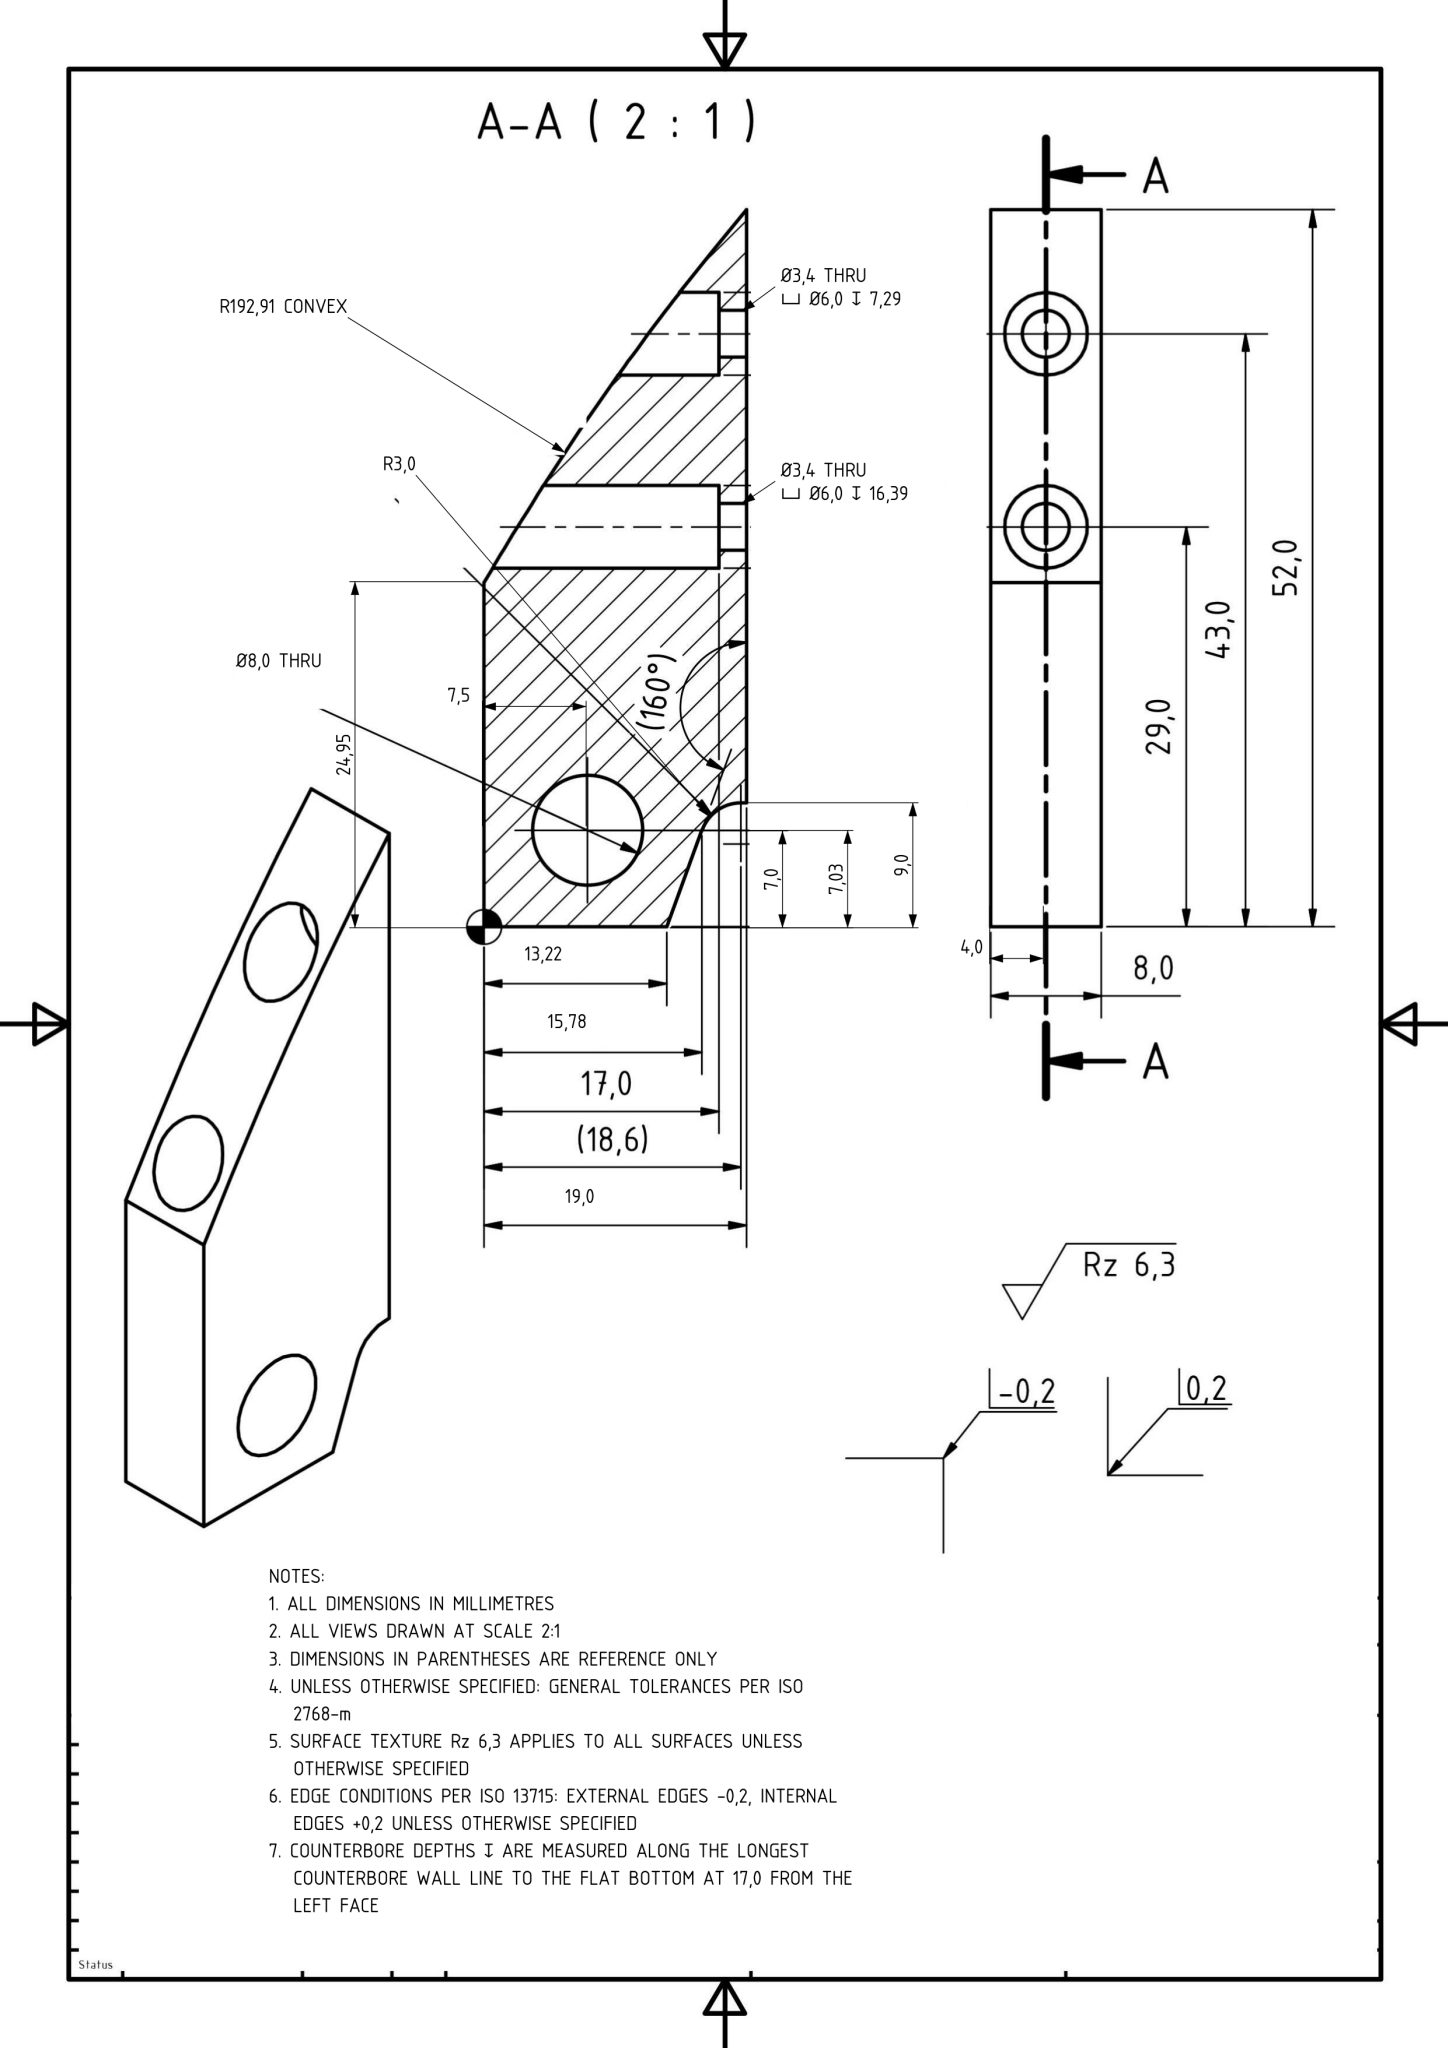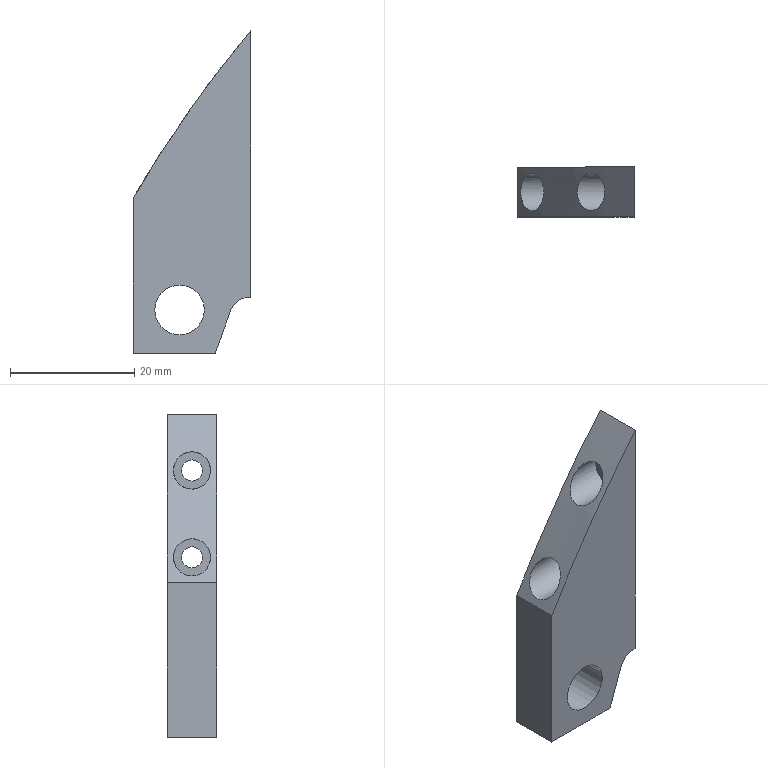Part | NX | mm | 1 solid | 16 faces | box 19 x 8 x 52 mm | volume 4687 mm3 | plane 9 | cylinder 7 | commonest cylinder face diameters 6 x3 3.4 x2 8 x1 385.82 x1
STEP:
#1=(LENGTH_UNIT()NAMED_UNIT(*)SI_UNIT(.MILLI.,.METRE.));
#2=UNCERTAINTY_MEASURE_WITH_UNIT(LENGTH_MEASURE(0.000001),#1,'','');
#3=(NAMED_UNIT(*)PLANE_ANGLE_UNIT()SI_UNIT($,.RADIAN.));
#4=PLANE_ANGLE_MEASURE_WITH_UNIT(PLANE_ANGLE_MEASURE(0.01745),#3);
#5=DIMENSIONAL_EXPONENTS(0.,0.,0.,0.,0.,0.,0.);
#6=(CONVERSION_BASED_UNIT('',#4)NAMED_UNIT(#5)PLANE_ANGLE_UNIT());
#7=(NAMED_UNIT(*)SI_UNIT($,.STERADIAN.)SOLID_ANGLE_UNIT());
#8=(GEOMETRIC_REPRESENTATION_CONTEXT(3)GLOBAL_UNCERTAINTY_ASSIGNED_CONTEXT((#2))GLOBAL_UNIT_ASSIGNED_CONTEXT((#6,#7,#1))REPRESENTATION_CONTEXT('',''));
#9=COLOUR_RGB('',0.898,0.9,0.9);
#10=FILL_AREA_STYLE_COLOUR('',#9);
#11=FILL_AREA_STYLE('',(#10));
#12=SURFACE_STYLE_FILL_AREA(#11);
#13=SURFACE_SIDE_STYLE('',(#12));
#14=SURFACE_STYLE_USAGE(.BOTH.,#13);
#15=PRESENTATION_STYLE_ASSIGNMENT((#14));
#16=CARTESIAN_POINT('',(-34.399,0.,-43.));
#17=VERTEX_POINT('',#16);
#18=CARTESIAN_POINT('',(-37.218,0.,-44.974));
#19=VERTEX_POINT('',#18);
#20=CARTESIAN_POINT('',(-34.399,0.,-46.));
#21=DIRECTION('',(0.,-1.,0.));
#22=DIRECTION('',(-0.5736,0.,0.8192));
#23=AXIS2_PLACEMENT_3D('',#20,#21,#22);
#24=CIRCLE('',#23,3.);
#25=EDGE_CURVE('',#17,#19,#24,.T.);
#26=ORIENTED_EDGE('',*,*,#25,.T.);
#27=CARTESIAN_POINT('',(-37.218,8.,-44.974));
#28=VERTEX_POINT('',#27);
#29=CARTESIAN_POINT('',(-37.218,0.,-44.974));
#30=DIRECTION('',(0.,1.,0.));
#31=VECTOR('',#30,8.);
#32=LINE('',#29,#31);
#33=EDGE_CURVE('',#19,#28,#32,.T.);
#34=ORIENTED_EDGE('',*,*,#33,.T.);
#35=CARTESIAN_POINT('',(-34.399,8.,-43.));
#36=VERTEX_POINT('',#35);
#37=CARTESIAN_POINT('',(-34.399,8.,-46.));
#38=DIRECTION('',(0.,1.,0.));
#39=DIRECTION('',(-0.5736,0.,0.8192));
#40=AXIS2_PLACEMENT_3D('',#37,#38,#39);
#41=CIRCLE('',#40,3.);
#42=EDGE_CURVE('',#28,#36,#41,.T.);
#43=ORIENTED_EDGE('',*,*,#42,.T.);
#44=CARTESIAN_POINT('',(-34.399,8.,-43.));
#45=DIRECTION('',(0.,-1.,0.));
#46=VECTOR('',#45,8.);
#47=LINE('',#44,#46);
#48=EDGE_CURVE('',#36,#17,#47,.T.);
#49=ORIENTED_EDGE('',*,*,#48,.T.);
#50=EDGE_LOOP('',(#26,#34,#43,#49));
#51=FACE_OUTER_BOUND('',#50,.T.);
#52=CARTESIAN_POINT('',(-34.399,0.,-46.));
#53=DIRECTION('',(0.,1.,0.));
#54=DIRECTION('',(-0.5736,0.,0.8192));
#55=AXIS2_PLACEMENT_3D('',#52,#53,#54);
#56=CYLINDRICAL_SURFACE('',#55,3.);
#57=ADVANCED_FACE('',(#51),#56,.F.);
#58=ORIENTED_EDGE('',*,*,#33,.F.);
#59=CARTESIAN_POINT('',(-39.776,0.,-52.));
#60=VERTEX_POINT('',#59);
#61=CARTESIAN_POINT('',(-37.218,0.,-44.974));
#62=DIRECTION('',(-0.342,0.,-0.9397));
#63=VECTOR('',#62,7.477);
#64=LINE('',#61,#63);
#65=EDGE_CURVE('',#19,#60,#64,.T.);
#66=ORIENTED_EDGE('',*,*,#65,.T.);
#67=CARTESIAN_POINT('',(-39.776,8.,-52.));
#68=VERTEX_POINT('',#67);
#69=CARTESIAN_POINT('',(-39.776,0.,-52.));
#70=DIRECTION('',(0.,1.,0.));
#71=VECTOR('',#70,8.);
#72=LINE('',#69,#71);
#73=EDGE_CURVE('',#60,#68,#72,.T.);
#74=ORIENTED_EDGE('',*,*,#73,.T.);
#75=CARTESIAN_POINT('',(-37.218,8.,-44.974));
#76=DIRECTION('',(-0.342,0.,-0.9397));
#77=VECTOR('',#76,7.477);
#78=LINE('',#75,#77);
#79=EDGE_CURVE('',#28,#68,#78,.T.);
#80=ORIENTED_EDGE('',*,*,#79,.F.);
#81=EDGE_LOOP('',(#58,#66,#74,#80));
#82=FACE_OUTER_BOUND('',#81,.T.);
#83=CARTESIAN_POINT('',(-36.5,0.,-43.));
#84=DIRECTION('',(0.9397,0.,-0.342));
#85=DIRECTION('',(-0.342,0.,-0.9397));
#86=AXIS2_PLACEMENT_3D('',#83,#84,#85);
#87=PLANE('',#86);
#88=ADVANCED_FACE('',(#82),#87,.T.);
#89=CARTESIAN_POINT('',(-43.29,4.,-12.));
#90=VERTEX_POINT('',#89);
#91=CARTESIAN_POINT('',(-43.29,4.,-12.));
#92=CARTESIAN_POINT('',(-43.29,4.373,-12.));
#93=CARTESIAN_POINT('',(-43.237,4.764,-11.926));
#94=CARTESIAN_POINT('',(-43.035,5.47,-11.643));
#95=CARTESIAN_POINT('',(-42.885,5.785,-11.435));
#96=CARTESIAN_POINT('',(-42.515,6.344,-10.92));
#97=CARTESIAN_POINT('',(-42.254,6.596,-10.56));
#98=CARTESIAN_POINT('',(-41.691,6.924,-9.79));
#99=CARTESIAN_POINT('',(-41.389,7.,-9.379));
#100=CARTESIAN_POINT('',(-40.822,7.,-8.616));
#101=CARTESIAN_POINT('',(-40.513,6.923,-8.203));
#102=CARTESIAN_POINT('',(-39.931,6.592,-7.432));
#103=CARTESIAN_POINT('',(-39.658,6.339,-7.073));
#104=CARTESIAN_POINT('',(-39.267,5.78,-6.563));
#105=CARTESIAN_POINT('',(-39.108,5.467,-6.356));
#106=CARTESIAN_POINT('',(-38.891,4.764,-6.074));
#107=CARTESIAN_POINT('',(-38.834,4.374,-6.));
#108=CARTESIAN_POINT('',(-38.834,3.626,-6.));
#109=CARTESIAN_POINT('',(-38.891,3.236,-6.074));
#110=CARTESIAN_POINT('',(-39.108,2.533,-6.356));
#111=CARTESIAN_POINT('',(-39.267,2.22,-6.563));
#112=CARTESIAN_POINT('',(-39.658,1.661,-7.073));
#113=CARTESIAN_POINT('',(-39.931,1.408,-7.432));
#114=CARTESIAN_POINT('',(-40.513,1.077,-8.203));
#115=CARTESIAN_POINT('',(-40.822,1.,-8.616));
#116=CARTESIAN_POINT('',(-41.389,1.,-9.379));
#117=CARTESIAN_POINT('',(-41.691,1.076,-9.79));
#118=CARTESIAN_POINT('',(-42.254,1.404,-10.56));
#119=CARTESIAN_POINT('',(-42.515,1.656,-10.92));
#120=CARTESIAN_POINT('',(-42.885,2.215,-11.435));
#121=CARTESIAN_POINT('',(-43.035,2.53,-11.643));
#122=CARTESIAN_POINT('',(-43.237,3.236,-11.926));
#123=CARTESIAN_POINT('',(-43.29,3.627,-12.));
#124=CARTESIAN_POINT('',(-43.29,4.,-12.));
#125=B_SPLINE_CURVE_WITH_KNOTS('',3,(#91,#92,#93,#94,#95,#96,#97,#98,#99,#100,#101,#102,#103,#104,#105,#106,#107,#108,#109,#110,#111,#112,#113,#114,#115,#116,#117,#118,#119,#120,#121,#122,#123,#124),.UNSPECIFIED.,.T.,.U.,(4,2,2,2,2,2,2,2,2,2,2,2,2,2,2,2,4),(0.,0.1119,0.2237,0.3655,0.5073,0.6507,0.7941,0.9062,1.018,1.13,1.243,1.386,1.529,1.671,1.813,1.925,2.037),.UNSPECIFIED.);
#126=EDGE_CURVE('',#90,#90,#125,.T.);
#127=ORIENTED_EDGE('',*,*,#126,.F.);
#128=EDGE_LOOP('',(#127));
#129=FACE_OUTER_BOUND('',#128,.T.);
#130=CARTESIAN_POINT('',(-36.,4.,-6.));
#131=VERTEX_POINT('',#130);
#132=CARTESIAN_POINT('',(-36.,4.,-9.));
#133=DIRECTION('',(1.,0.,0.));
#134=DIRECTION('',(0.,0.,-1.));
#135=AXIS2_PLACEMENT_3D('',#132,#133,#134);
#136=CIRCLE('',#135,3.);
#137=EDGE_CURVE('',#131,#131,#136,.T.);
#138=ORIENTED_EDGE('',*,*,#137,.T.);
#139=EDGE_LOOP('',(#138));
#140=FACE_BOUND('',#139,.T.);
#141=CARTESIAN_POINT('',(-53.,4.,-9.));
#142=DIRECTION('',(1.,0.,-0.));
#143=DIRECTION('',(0.,0.,-1.));
#144=AXIS2_PLACEMENT_3D('',#141,#142,#143);
#145=CYLINDRICAL_SURFACE('',#144,3.);
#146=ADVANCED_FACE('',(#129,#140),#145,.F.);
#147=ORIENTED_EDGE('',*,*,#137,.F.);
#148=EDGE_LOOP('',(#147));
#149=FACE_OUTER_BOUND('',#148,.T.);
#150=CARTESIAN_POINT('',(-36.,4.,-10.7));
#151=VERTEX_POINT('',#150);
#152=CARTESIAN_POINT('',(-36.,4.,-9.));
#153=DIRECTION('',(-1.,0.,0.));
#154=DIRECTION('',(0.,0.,-1.));
#155=AXIS2_PLACEMENT_3D('',#152,#153,#154);
#156=CIRCLE('',#155,1.7);
#157=EDGE_CURVE('',#151,#151,#156,.T.);
#158=ORIENTED_EDGE('',*,*,#157,.F.);
#159=EDGE_LOOP('',(#158));
#160=FACE_BOUND('',#159,.T.);
#161=CARTESIAN_POINT('',(-36.,4.,-9.));
#162=DIRECTION('',(1.,0.,0.));
#163=DIRECTION('',(0.,0.,-1.));
#164=AXIS2_PLACEMENT_3D('',#161,#162,#163);
#165=PLANE('',#164);
#166=ADVANCED_FACE('',(#149,#160),#165,.F.);
#167=CARTESIAN_POINT('',(-52.386,4.,-26.));
#168=VERTEX_POINT('',#167);
#169=CARTESIAN_POINT('',(-52.386,4.,-26.));
#170=CARTESIAN_POINT('',(-52.386,4.374,-26.));
#171=CARTESIAN_POINT('',(-52.342,4.768,-25.926));
#172=CARTESIAN_POINT('',(-52.171,5.483,-25.636));
#173=CARTESIAN_POINT('',(-52.043,5.804,-25.422));
#174=CARTESIAN_POINT('',(-51.734,6.356,-24.903));
#175=CARTESIAN_POINT('',(-51.522,6.602,-24.549));
#176=CARTESIAN_POINT('',(-51.061,6.924,-23.787));
#177=CARTESIAN_POINT('',(-50.812,7.,-23.379));
#178=CARTESIAN_POINT('',(-50.345,7.,-22.618));
#179=CARTESIAN_POINT('',(-50.091,6.923,-22.208));
#180=CARTESIAN_POINT('',(-49.614,6.599,-21.445));
#181=CARTESIAN_POINT('',(-49.392,6.351,-21.092));
#182=CARTESIAN_POINT('',(-49.065,5.801,-20.576));
#183=CARTESIAN_POINT('',(-48.929,5.481,-20.363));
#184=CARTESIAN_POINT('',(-48.745,4.768,-20.075));
#185=CARTESIAN_POINT('',(-48.698,4.374,-20.));
#186=CARTESIAN_POINT('',(-48.698,3.626,-20.));
#187=CARTESIAN_POINT('',(-48.745,3.232,-20.075));
#188=CARTESIAN_POINT('',(-48.929,2.519,-20.363));
#189=CARTESIAN_POINT('',(-49.065,2.199,-20.576));
#190=CARTESIAN_POINT('',(-49.392,1.649,-21.092));
#191=CARTESIAN_POINT('',(-49.614,1.401,-21.445));
#192=CARTESIAN_POINT('',(-50.091,1.077,-22.208));
#193=CARTESIAN_POINT('',(-50.345,1.,-22.618));
#194=CARTESIAN_POINT('',(-50.812,1.,-23.379));
#195=CARTESIAN_POINT('',(-51.061,1.076,-23.787));
#196=CARTESIAN_POINT('',(-51.522,1.398,-24.549));
#197=CARTESIAN_POINT('',(-51.734,1.644,-24.903));
#198=CARTESIAN_POINT('',(-52.043,2.196,-25.422));
#199=CARTESIAN_POINT('',(-52.171,2.517,-25.636));
#200=CARTESIAN_POINT('',(-52.342,3.232,-25.926));
#201=CARTESIAN_POINT('',(-52.386,3.626,-26.));
#202=CARTESIAN_POINT('',(-52.386,4.,-26.));
#203=B_SPLINE_CURVE_WITH_KNOTS('',3,(#169,#170,#171,#172,#173,#174,#175,#176,#177,#178,#179,#180,#181,#182,#183,#184,#185,#186,#187,#188,#189,#190,#191,#192,#193,#194,#195,#196,#197,#198,#199,#200,#201,#202),.UNSPECIFIED.,.T.,.U.,(4,2,2,2,2,2,2,2,2,2,2,2,2,2,2,2,4),(0.,0.1121,0.2242,0.3575,0.4908,0.6253,0.7597,0.872,0.9843,1.097,1.209,1.343,1.478,1.611,1.744,1.856,1.969),.UNSPECIFIED.);
#204=EDGE_CURVE('',#168,#168,#203,.T.);
#205=ORIENTED_EDGE('',*,*,#204,.F.);
#206=EDGE_LOOP('',(#205));
#207=FACE_OUTER_BOUND('',#206,.T.);
#208=CARTESIAN_POINT('',(-36.,4.,-20.));
#209=VERTEX_POINT('',#208);
#210=CARTESIAN_POINT('',(-36.,4.,-23.));
#211=DIRECTION('',(1.,0.,0.));
#212=DIRECTION('',(0.,0.,-1.));
#213=AXIS2_PLACEMENT_3D('',#210,#211,#212);
#214=CIRCLE('',#213,3.);
#215=EDGE_CURVE('',#209,#209,#214,.T.);
#216=ORIENTED_EDGE('',*,*,#215,.T.);
#217=EDGE_LOOP('',(#216));
#218=FACE_BOUND('',#217,.T.);
#219=CARTESIAN_POINT('',(-53.,4.,-23.));
#220=DIRECTION('',(1.,0.,-0.));
#221=DIRECTION('',(0.,0.,-1.));
#222=AXIS2_PLACEMENT_3D('',#219,#220,#221);
#223=CYLINDRICAL_SURFACE('',#222,3.);
#224=ADVANCED_FACE('',(#207,#218),#223,.F.);
#225=ORIENTED_EDGE('',*,*,#215,.F.);
#226=EDGE_LOOP('',(#225));
#227=FACE_OUTER_BOUND('',#226,.T.);
#228=CARTESIAN_POINT('',(-36.,4.,-21.3));
#229=VERTEX_POINT('',#228);
#230=CARTESIAN_POINT('',(-36.,4.,-23.));
#231=DIRECTION('',(-1.,0.,0.));
#232=DIRECTION('',(0.,0.,-1.));
#233=AXIS2_PLACEMENT_3D('',#230,#231,#232);
#234=CIRCLE('',#233,1.7);
#235=EDGE_CURVE('',#229,#229,#234,.T.);
#236=ORIENTED_EDGE('',*,*,#235,.F.);
#237=EDGE_LOOP('',(#236));
#238=FACE_BOUND('',#237,.T.);
#239=CARTESIAN_POINT('',(-36.,4.,-23.));
#240=DIRECTION('',(1.,0.,0.));
#241=DIRECTION('',(0.,0.,-1.));
#242=AXIS2_PLACEMENT_3D('',#239,#240,#241);
#243=PLANE('',#242);
#244=ADVANCED_FACE('',(#227,#238),#243,.F.);
#245=ORIENTED_EDGE('',*,*,#157,.T.);
#246=EDGE_LOOP('',(#245));
#247=FACE_OUTER_BOUND('',#246,.T.);
#248=CARTESIAN_POINT('',(-34.,4.,-10.7));
#249=VERTEX_POINT('',#248);
#250=CARTESIAN_POINT('',(-34.,4.,-9.));
#251=DIRECTION('',(-1.,0.,0.));
#252=DIRECTION('',(0.,0.,-1.));
#253=AXIS2_PLACEMENT_3D('',#250,#251,#252);
#254=CIRCLE('',#253,1.7);
#255=EDGE_CURVE('',#249,#249,#254,.T.);
#256=ORIENTED_EDGE('',*,*,#255,.F.);
#257=EDGE_LOOP('',(#256));
#258=FACE_BOUND('',#257,.T.);
#259=CARTESIAN_POINT('',(-89.937,4.,-9.));
#260=DIRECTION('',(1.,0.,-0.));
#261=DIRECTION('',(0.,0.,-1.));
#262=AXIS2_PLACEMENT_3D('',#259,#260,#261);
#263=CYLINDRICAL_SURFACE('',#262,1.7);
#264=ADVANCED_FACE('',(#247,#258),#263,.F.);
#265=ORIENTED_EDGE('',*,*,#235,.T.);
#266=EDGE_LOOP('',(#265));
#267=FACE_OUTER_BOUND('',#266,.T.);
#268=CARTESIAN_POINT('',(-34.,4.,-24.7));
#269=VERTEX_POINT('',#268);
#270=CARTESIAN_POINT('',(-34.,4.,-23.));
#271=DIRECTION('',(-1.,0.,0.));
#272=DIRECTION('',(0.,0.,-1.));
#273=AXIS2_PLACEMENT_3D('',#270,#271,#272);
#274=CIRCLE('',#273,1.7);
#275=EDGE_CURVE('',#269,#269,#274,.T.);
#276=ORIENTED_EDGE('',*,*,#275,.F.);
#277=EDGE_LOOP('',(#276));
#278=FACE_BOUND('',#277,.T.);
#279=CARTESIAN_POINT('',(-89.937,4.,-23.));
#280=DIRECTION('',(1.,0.,-0.));
#281=DIRECTION('',(0.,0.,-1.));
#282=AXIS2_PLACEMENT_3D('',#279,#280,#281);
#283=CYLINDRICAL_SURFACE('',#282,1.7);
#284=ADVANCED_FACE('',(#267,#278),#283,.F.);
#285=CARTESIAN_POINT('',(-49.5,8.,-45.));
#286=VERTEX_POINT('',#285);
#287=CARTESIAN_POINT('',(-45.5,8.,-45.));
#288=DIRECTION('',(0.,-1.,0.));
#289=DIRECTION('',(1.,0.,0.));
#290=AXIS2_PLACEMENT_3D('',#287,#288,#289);
#291=CIRCLE('',#290,4.);
#292=EDGE_CURVE('',#286,#286,#291,.T.);
#293=ORIENTED_EDGE('',*,*,#292,.F.);
#294=EDGE_LOOP('',(#293));
#295=FACE_OUTER_BOUND('',#294,.T.);
#296=CARTESIAN_POINT('',(-49.5,0.,-45.));
#297=VERTEX_POINT('',#296);
#298=CARTESIAN_POINT('',(-45.5,0.,-45.));
#299=DIRECTION('',(0.,1.,0.));
#300=DIRECTION('',(1.,0.,0.));
#301=AXIS2_PLACEMENT_3D('',#298,#299,#300);
#302=CIRCLE('',#301,4.);
#303=EDGE_CURVE('',#297,#297,#302,.T.);
#304=ORIENTED_EDGE('',*,*,#303,.F.);
#305=EDGE_LOOP('',(#304));
#306=FACE_BOUND('',#305,.T.);
#307=CARTESIAN_POINT('',(-45.5,0.,-45.));
#308=DIRECTION('',(0.,1.,0.));
#309=DIRECTION('',(1.,0.,0.));
#310=AXIS2_PLACEMENT_3D('',#307,#308,#309);
#311=CYLINDRICAL_SURFACE('',#310,4.);
#312=ADVANCED_FACE('',(#295,#306),#311,.F.);
#313=CARTESIAN_POINT('',(-53.,0.,-27.049));
#314=VERTEX_POINT('',#313);
#315=CARTESIAN_POINT('',(-34.,0.,0.));
#316=VERTEX_POINT('',#315);
#317=CARTESIAN_POINT('',(113.777,0.,-124.));
#318=DIRECTION('',(0.,1.,0.));
#319=DIRECTION('',(-0.8645,0.,0.5026));
#320=AXIS2_PLACEMENT_3D('',#317,#318,#319);
#321=CIRCLE('',#320,192.91);
#322=EDGE_CURVE('',#314,#316,#321,.T.);
#323=ORIENTED_EDGE('',*,*,#322,.T.);
#324=CARTESIAN_POINT('',(-34.,8.,0.));
#325=VERTEX_POINT('',#324);
#326=CARTESIAN_POINT('',(-34.,0.,0.));
#327=DIRECTION('',(0.,1.,0.));
#328=VECTOR('',#327,8.);
#329=LINE('',#326,#328);
#330=EDGE_CURVE('',#316,#325,#329,.T.);
#331=ORIENTED_EDGE('',*,*,#330,.T.);
#332=CARTESIAN_POINT('',(-53.,8.,-27.049));
#333=VERTEX_POINT('',#332);
#334=CARTESIAN_POINT('',(113.777,8.,-124.));
#335=DIRECTION('',(0.,1.,0.));
#336=DIRECTION('',(-0.8645,0.,0.5026));
#337=AXIS2_PLACEMENT_3D('',#334,#335,#336);
#338=CIRCLE('',#337,192.91);
#339=EDGE_CURVE('',#333,#325,#338,.T.);
#340=ORIENTED_EDGE('',*,*,#339,.F.);
#341=CARTESIAN_POINT('',(-53.,0.,-27.049));
#342=DIRECTION('',(0.,1.,0.));
#343=VECTOR('',#342,8.);
#344=LINE('',#341,#343);
#345=EDGE_CURVE('',#314,#333,#344,.T.);
#346=ORIENTED_EDGE('',*,*,#345,.F.);
#347=EDGE_LOOP('',(#323,#331,#340,#346));
#348=FACE_OUTER_BOUND('',#347,.T.);
#349=ORIENTED_EDGE('',*,*,#126,.T.);
#350=EDGE_LOOP('',(#349));
#351=FACE_BOUND('',#350,.T.);
#352=ORIENTED_EDGE('',*,*,#204,.T.);
#353=EDGE_LOOP('',(#352));
#354=FACE_BOUND('',#353,.T.);
#355=CARTESIAN_POINT('',(113.777,0.,-124.));
#356=DIRECTION('',(0.,1.,0.));
#357=DIRECTION('',(-0.8645,0.,0.5026));
#358=AXIS2_PLACEMENT_3D('',#355,#356,#357);
#359=CYLINDRICAL_SURFACE('',#358,192.91);
#360=ADVANCED_FACE('',(#348,#351,#354),#359,.T.);
#361=CARTESIAN_POINT('',(-53.,0.,-52.));
#362=VERTEX_POINT('',#361);
#363=CARTESIAN_POINT('',(-53.,0.,-52.));
#364=DIRECTION('',(0.,0.,1.));
#365=VECTOR('',#364,24.951);
#366=LINE('',#363,#365);
#367=EDGE_CURVE('',#362,#314,#366,.T.);
#368=ORIENTED_EDGE('',*,*,#367,.T.);
#369=ORIENTED_EDGE('',*,*,#345,.T.);
#370=CARTESIAN_POINT('',(-53.,8.,-52.));
#371=VERTEX_POINT('',#370);
#372=CARTESIAN_POINT('',(-53.,8.,-52.));
#373=DIRECTION('',(0.,0.,1.));
#374=VECTOR('',#373,24.951);
#375=LINE('',#372,#374);
#376=EDGE_CURVE('',#371,#333,#375,.T.);
#377=ORIENTED_EDGE('',*,*,#376,.F.);
#378=CARTESIAN_POINT('',(-53.,0.,-52.));
#379=DIRECTION('',(0.,1.,0.));
#380=VECTOR('',#379,8.);
#381=LINE('',#378,#380);
#382=EDGE_CURVE('',#362,#371,#381,.T.);
#383=ORIENTED_EDGE('',*,*,#382,.F.);
#384=EDGE_LOOP('',(#368,#369,#377,#383));
#385=FACE_OUTER_BOUND('',#384,.T.);
#386=CARTESIAN_POINT('',(-53.,0.,-52.));
#387=DIRECTION('',(-1.,0.,0.));
#388=DIRECTION('',(0.,0.,1.));
#389=AXIS2_PLACEMENT_3D('',#386,#387,#388);
#390=PLANE('',#389);
#391=ADVANCED_FACE('',(#385),#390,.T.);
#392=CARTESIAN_POINT('',(-39.776,0.,-52.));
#393=DIRECTION('',(-1.,0.,0.));
#394=VECTOR('',#393,13.224);
#395=LINE('',#392,#394);
#396=EDGE_CURVE('',#60,#362,#395,.T.);
#397=ORIENTED_EDGE('',*,*,#396,.T.);
#398=ORIENTED_EDGE('',*,*,#382,.T.);
#399=CARTESIAN_POINT('',(-39.776,8.,-52.));
#400=DIRECTION('',(-1.,0.,0.));
#401=VECTOR('',#400,13.224);
#402=LINE('',#399,#401);
#403=EDGE_CURVE('',#68,#371,#402,.T.);
#404=ORIENTED_EDGE('',*,*,#403,.F.);
#405=ORIENTED_EDGE('',*,*,#73,.F.);
#406=EDGE_LOOP('',(#397,#398,#404,#405));
#407=FACE_OUTER_BOUND('',#406,.T.);
#408=CARTESIAN_POINT('',(-39.776,0.,-52.));
#409=DIRECTION('',(0.,0.,-1.));
#410=DIRECTION('',(-1.,0.,0.));
#411=AXIS2_PLACEMENT_3D('',#408,#409,#410);
#412=PLANE('',#411);
#413=ADVANCED_FACE('',(#407),#412,.T.);
#414=ORIENTED_EDGE('',*,*,#48,.F.);
#415=CARTESIAN_POINT('',(-34.,8.,-43.));
#416=VERTEX_POINT('',#415);
#417=CARTESIAN_POINT('',(-34.,8.,-43.));
#418=DIRECTION('',(-1.,0.,0.));
#419=VECTOR('',#418,0.3994);
#420=LINE('',#417,#419);
#421=EDGE_CURVE('',#416,#36,#420,.T.);
#422=ORIENTED_EDGE('',*,*,#421,.F.);
#423=CARTESIAN_POINT('',(-34.,0.,-43.));
#424=VERTEX_POINT('',#423);
#425=CARTESIAN_POINT('',(-34.,0.,-43.));
#426=DIRECTION('',(0.,1.,0.));
#427=VECTOR('',#426,8.);
#428=LINE('',#425,#427);
#429=EDGE_CURVE('',#424,#416,#428,.T.);
#430=ORIENTED_EDGE('',*,*,#429,.F.);
#431=CARTESIAN_POINT('',(-34.,0.,-43.));
#432=DIRECTION('',(-1.,0.,0.));
#433=VECTOR('',#432,0.3994);
#434=LINE('',#431,#433);
#435=EDGE_CURVE('',#424,#17,#434,.T.);
#436=ORIENTED_EDGE('',*,*,#435,.T.);
#437=EDGE_LOOP('',(#414,#422,#430,#436));
#438=FACE_OUTER_BOUND('',#437,.T.);
#439=CARTESIAN_POINT('',(-34.,0.,-43.));
#440=DIRECTION('',(0.,0.,-1.));
#441=DIRECTION('',(-1.,0.,0.));
#442=AXIS2_PLACEMENT_3D('',#439,#440,#441);
#443=PLANE('',#442);
#444=ADVANCED_FACE('',(#438),#443,.T.);
#445=CARTESIAN_POINT('',(-34.,0.,0.));
#446=DIRECTION('',(0.,0.,-1.));
#447=VECTOR('',#446,43.);
#448=LINE('',#445,#447);
#449=EDGE_CURVE('',#316,#424,#448,.T.);
#450=ORIENTED_EDGE('',*,*,#449,.T.);
#451=ORIENTED_EDGE('',*,*,#429,.T.);
#452=CARTESIAN_POINT('',(-34.,8.,0.));
#453=DIRECTION('',(0.,0.,-1.));
#454=VECTOR('',#453,43.);
#455=LINE('',#452,#454);
#456=EDGE_CURVE('',#325,#416,#455,.T.);
#457=ORIENTED_EDGE('',*,*,#456,.F.);
#458=ORIENTED_EDGE('',*,*,#330,.F.);
#459=EDGE_LOOP('',(#450,#451,#457,#458));
#460=FACE_OUTER_BOUND('',#459,.T.);
#461=ORIENTED_EDGE('',*,*,#255,.T.);
#462=EDGE_LOOP('',(#461));
#463=FACE_BOUND('',#462,.T.);
#464=ORIENTED_EDGE('',*,*,#275,.T.);
#465=EDGE_LOOP('',(#464));
#466=FACE_BOUND('',#465,.T.);
#467=CARTESIAN_POINT('',(-34.,0.,0.));
#468=DIRECTION('',(1.,0.,0.));
#469=DIRECTION('',(0.,0.,-1.));
#470=AXIS2_PLACEMENT_3D('',#467,#468,#469);
#471=PLANE('',#470);
#472=ADVANCED_FACE('',(#460,#463,#466),#471,.T.);
#473=ORIENTED_EDGE('',*,*,#456,.T.);
#474=ORIENTED_EDGE('',*,*,#421,.T.);
#475=ORIENTED_EDGE('',*,*,#42,.F.);
#476=ORIENTED_EDGE('',*,*,#79,.T.);
#477=ORIENTED_EDGE('',*,*,#403,.T.);
#478=ORIENTED_EDGE('',*,*,#376,.T.);
#479=ORIENTED_EDGE('',*,*,#339,.T.);
#480=EDGE_LOOP('',(#473,#474,#475,#476,#477,#478,#479));
#481=FACE_OUTER_BOUND('',#480,.T.);
#482=ORIENTED_EDGE('',*,*,#292,.T.);
#483=EDGE_LOOP('',(#482));
#484=FACE_BOUND('',#483,.T.);
#485=CARTESIAN_POINT('',(-41.843,8.,-29.555));
#486=DIRECTION('',(0.,-1.,0.));
#487=DIRECTION('',(0.,0.,-1.));
#488=AXIS2_PLACEMENT_3D('',#485,#486,#487);
#489=PLANE('',#488);
#490=ADVANCED_FACE('',(#481,#484),#489,.F.);
#491=ORIENTED_EDGE('',*,*,#449,.F.);
#492=ORIENTED_EDGE('',*,*,#322,.F.);
#493=ORIENTED_EDGE('',*,*,#367,.F.);
#494=ORIENTED_EDGE('',*,*,#396,.F.);
#495=ORIENTED_EDGE('',*,*,#65,.F.);
#496=ORIENTED_EDGE('',*,*,#25,.F.);
#497=ORIENTED_EDGE('',*,*,#435,.F.);
#498=EDGE_LOOP('',(#491,#492,#493,#494,#495,#496,#497));
#499=FACE_OUTER_BOUND('',#498,.T.);
#500=ORIENTED_EDGE('',*,*,#303,.T.);
#501=EDGE_LOOP('',(#500));
#502=FACE_BOUND('',#501,.T.);
#503=CARTESIAN_POINT('',(-41.843,0.,-29.555));
#504=DIRECTION('',(0.,-1.,0.));
#505=DIRECTION('',(0.,0.,-1.));
#506=AXIS2_PLACEMENT_3D('',#503,#504,#505);
#507=PLANE('',#506);
#508=ADVANCED_FACE('',(#499,#502),#507,.T.);
#509=CLOSED_SHELL('',(#57,#88,#146,#166,#224,#244,#264,#284,#312,#360,#391,#413,#444,#472,#490,#508));
#510=MANIFOLD_SOLID_BREP('',#509);
#511=STYLED_ITEM('',(#15),#510);
#512=(LENGTH_UNIT()NAMED_UNIT(*)SI_UNIT(.MILLI.,.METRE.));
#513=UNCERTAINTY_MEASURE_WITH_UNIT(LENGTH_MEASURE(0.01),#512,'','');
#514=(NAMED_UNIT(*)PLANE_ANGLE_UNIT()SI_UNIT($,.RADIAN.));
#515=PLANE_ANGLE_MEASURE_WITH_UNIT(PLANE_ANGLE_MEASURE(0.01745),#514);
#516=DIMENSIONAL_EXPONENTS(0.,0.,0.,0.,0.,0.,0.);
#517=(CONVERSION_BASED_UNIT('',#515)NAMED_UNIT(#516)PLANE_ANGLE_UNIT());
#518=(NAMED_UNIT(*)SI_UNIT($,.STERADIAN.)SOLID_ANGLE_UNIT());
#519=(GEOMETRIC_REPRESENTATION_CONTEXT(3)GLOBAL_UNCERTAINTY_ASSIGNED_CONTEXT((#513))GLOBAL_UNIT_ASSIGNED_CONTEXT((#517,#518,#512))REPRESENTATION_CONTEXT('',''));
#520=MECHANICAL_DESIGN_GEOMETRIC_PRESENTATION_REPRESENTATION('',(#511),#519);
#521=ADVANCED_BREP_SHAPE_REPRESENTATION('',(#510),#519);
#522=CARTESIAN_POINT('',(0.,0.,0.));
#523=DIRECTION('',(0.,0.,1.));
#524=DIRECTION('',(1.,0.,0.));
#525=AXIS2_PLACEMENT_3D('',#522,#523,#524);
#526=SHAPE_REPRESENTATION('',(#525),#519);
#527=SHAPE_REPRESENTATION_RELATIONSHIP('','',#521,#526);